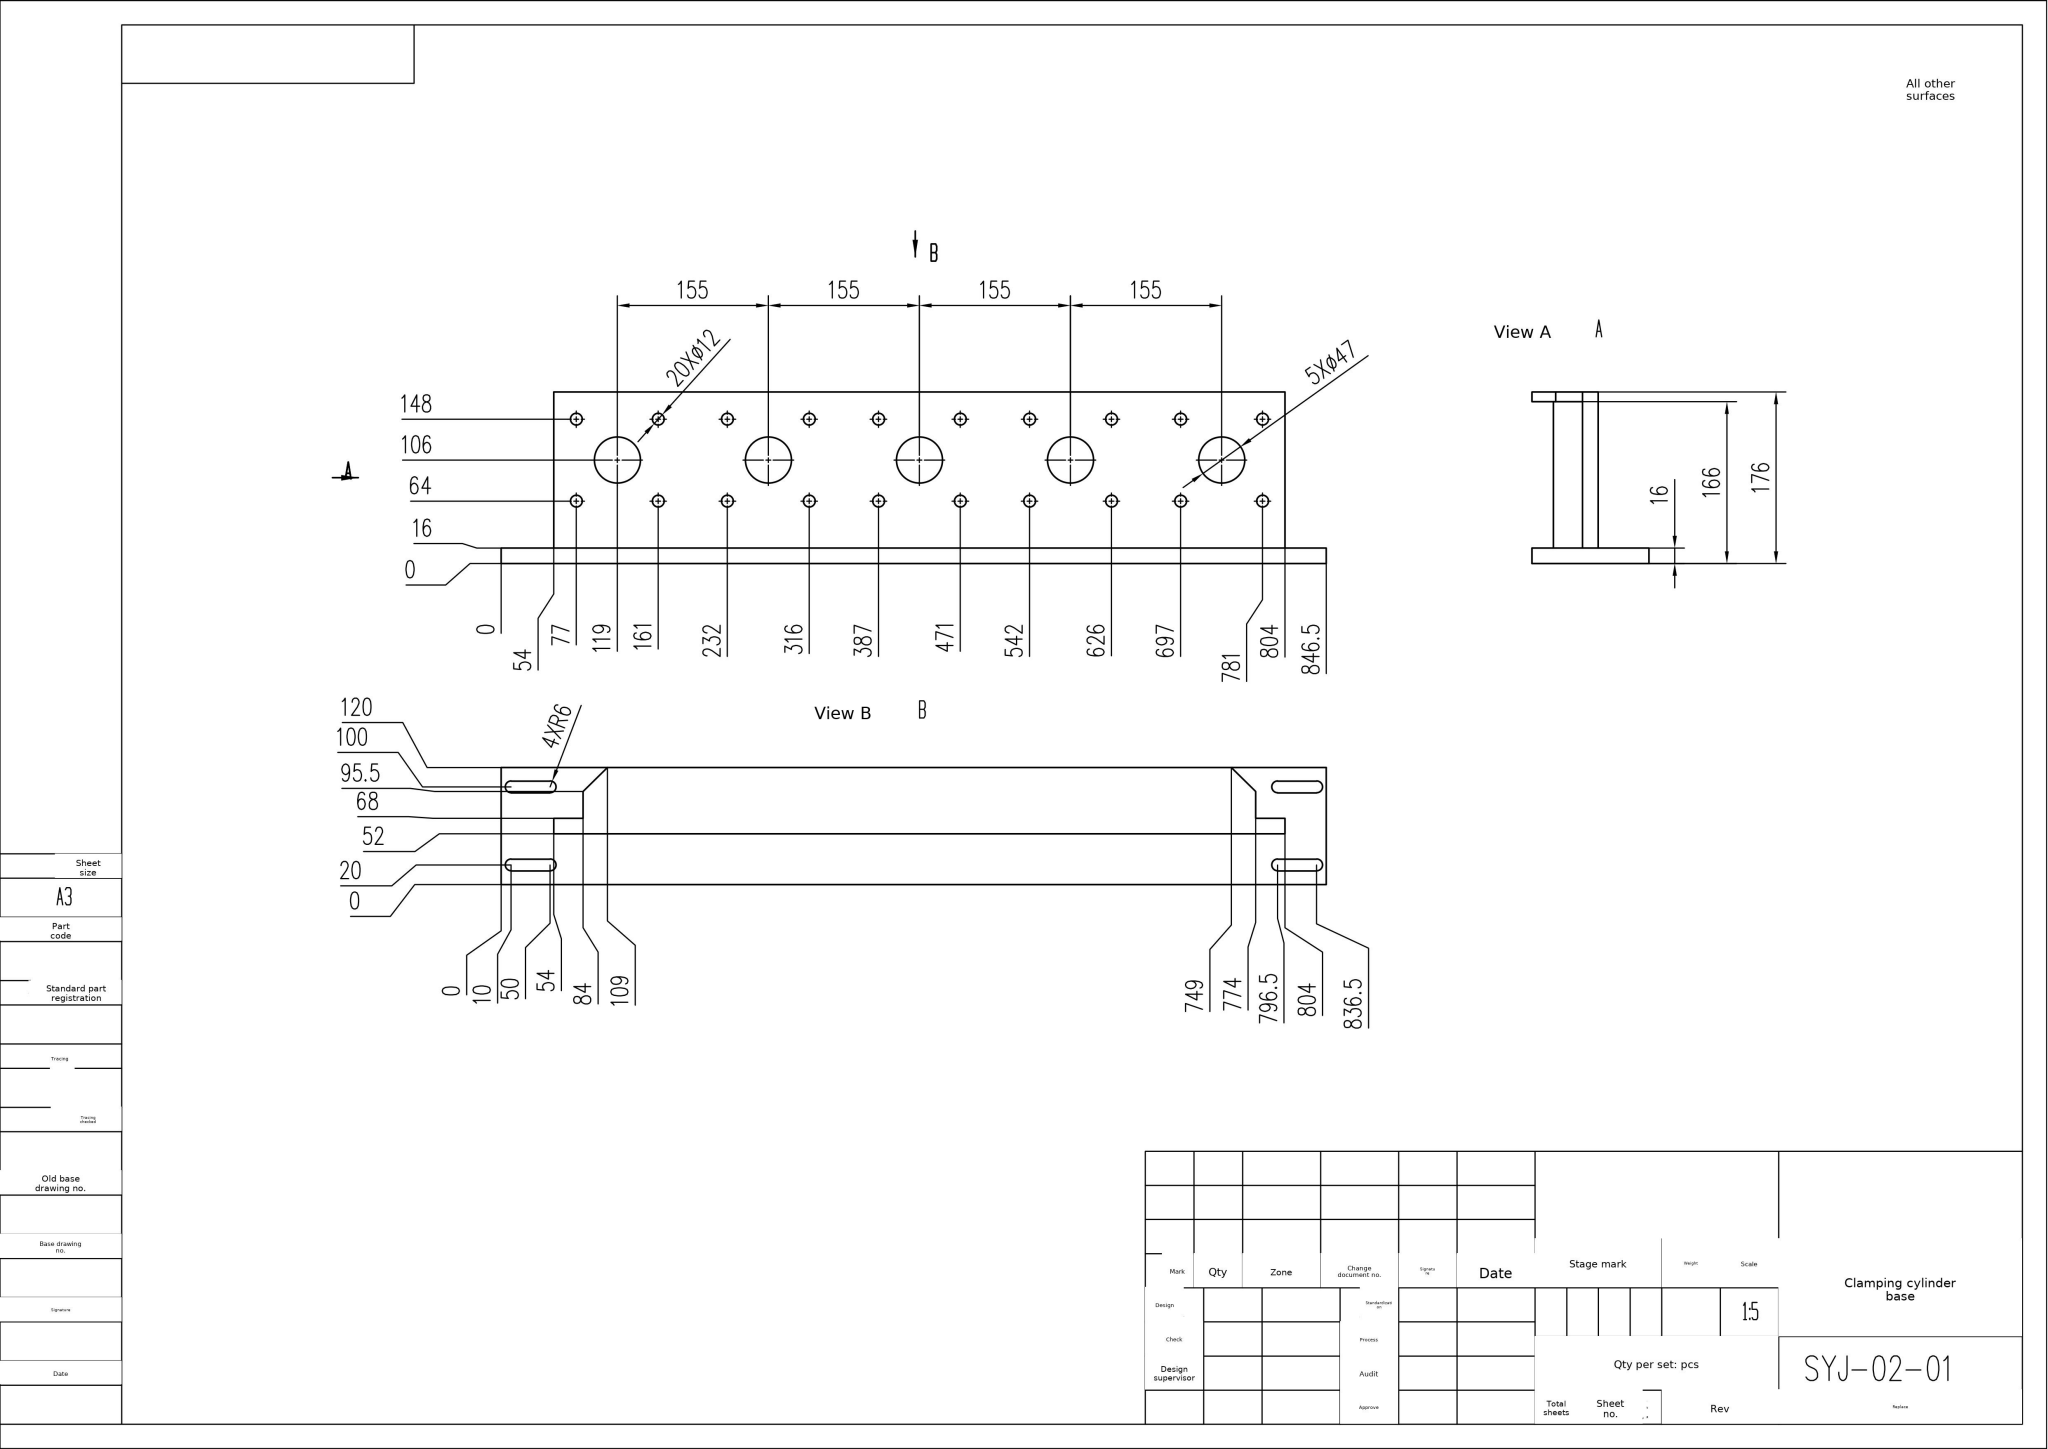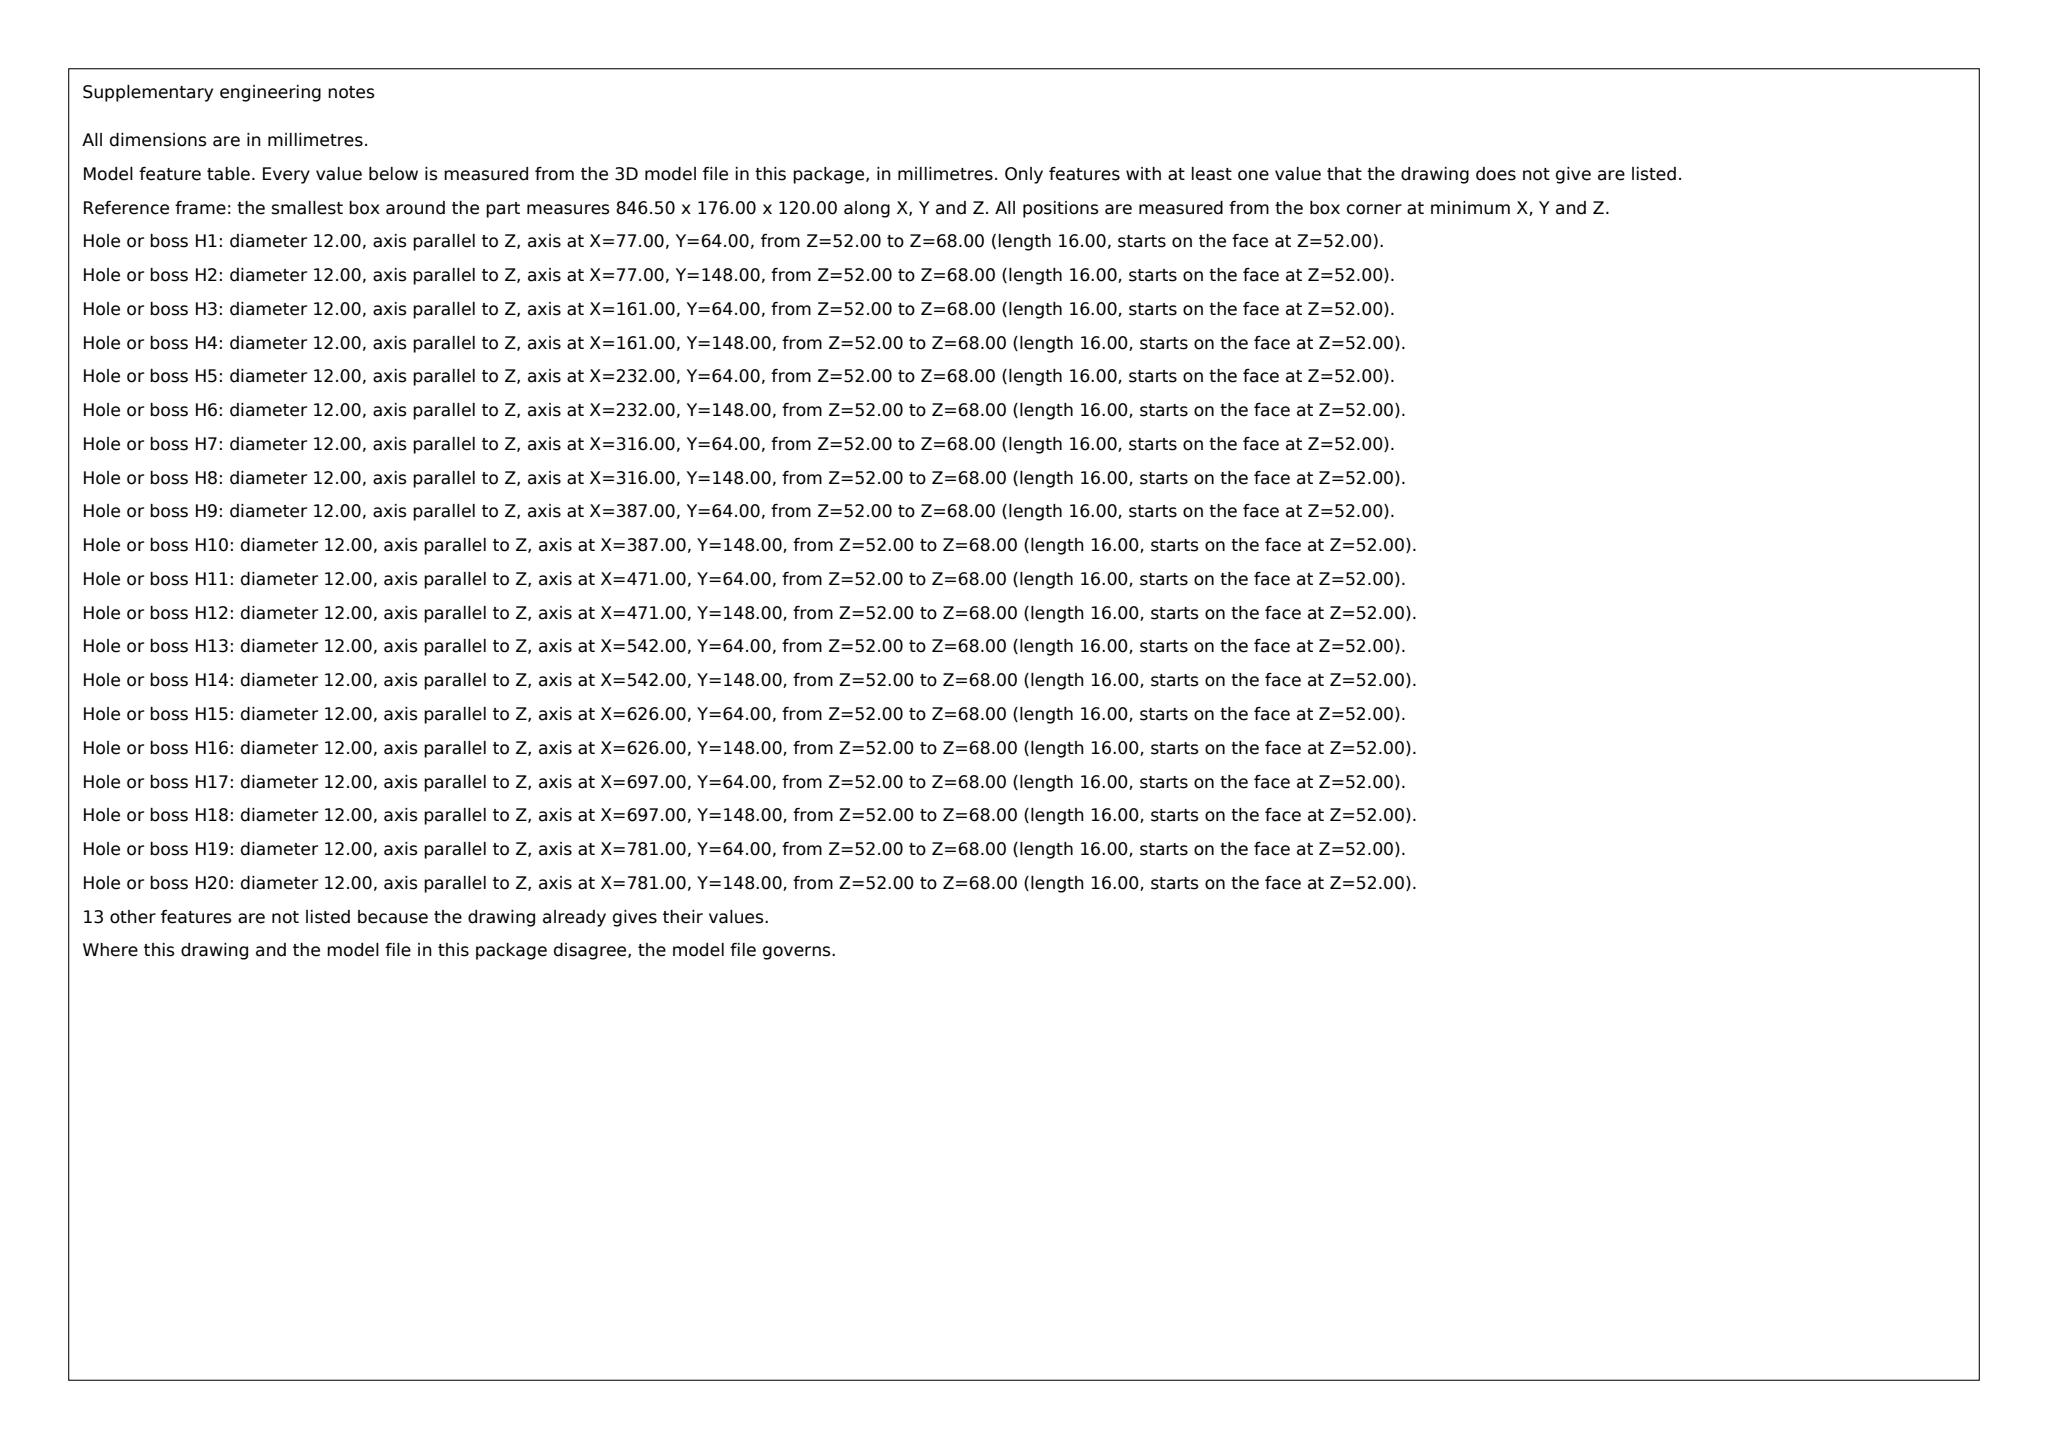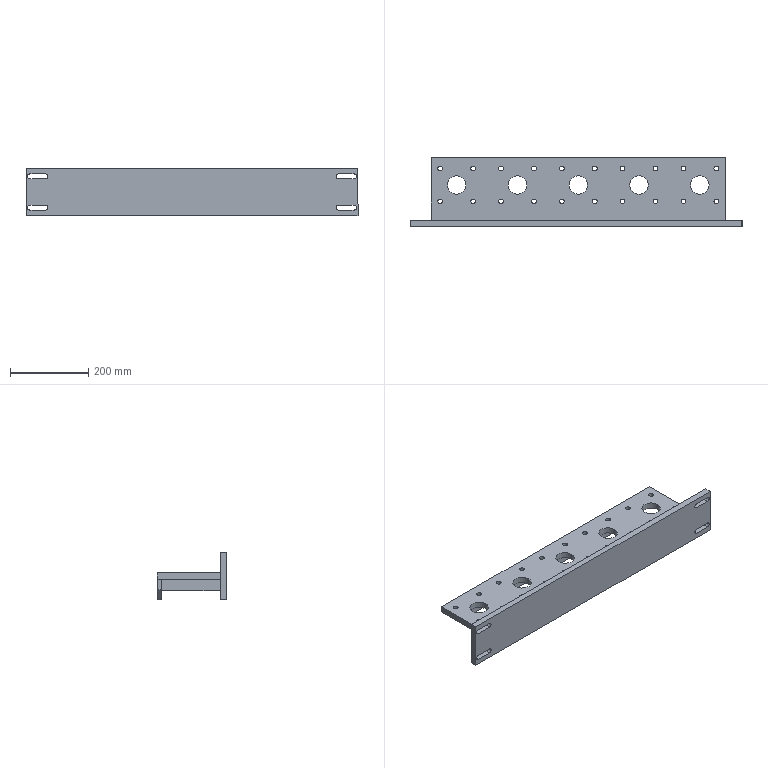Part | SolidWorks | mm | 1 solid | 91 faces | box 846.5 x 176 x 120 mm | volume 3739017 mm3 | cylinder 58 | plane 33 | commonest cylinder face diameters 12 x48 47 x10
build123d program:
from build123d import *

# Parameters (mm, degrees)
SKETCH1_W           = 810
SKETCH1_H           = 120
BOSS_EXTRUDE1_DEPTH = 16
SKETCH2_W           = 750
SKETCH2_H           = 16
BOSS_EXTRUDE2_DEPTH = 160
SKETCH5_W           = 750
SKETCH5_H           = 52
BOSS_EXTRUDE4_DEPTH = 10
CUT_EXTRUDE1_REACH  = 448.794
SKETCH6_R           = 23.5
CUT_EXTRUDE2_REACH  = 448.794
SKETCH7_R           = 6
CHAMFER1_SIZE       = 25
SKETCH9_W           = 120
SKETCH9_H           = 16
BOSS_EXTRUDE6_DEPTH = 12.5
SKETCH10_W          = 120
SKETCH10_H          = 16
BOSS_EXTRUDE7_DEPTH = 24
CUT_EXTRUDE3_DEPTH  = 16
CUT_EXTRUDE4_DEPTH  = 10
SKETCH15_W          = 6
SKETCH15_H          = 150
BOSS_EXTRUDE8_DEPTH = 30


with BuildPart() as part:
    # Sketch1 → Boss-Extrude1 (new body)
    with BuildSketch(Plane(origin=(0, 0, 0), x_dir=(1, 0, 0), z_dir=(0, 1, 0))):
        Rectangle(SKETCH1_W, SKETCH1_H)
    extrude(amount=BOSS_EXTRUDE1_DEPTH)

    # Sketch2 → Boss-Extrude2 (add)
    with BuildSketch(Plane(origin=(0, 16, 0), x_dir=(1, 0, 0), z_dir=(0, 1, 0))):
        Rectangle(SKETCH2_W, SKETCH2_H)
    extrude(amount=BOSS_EXTRUDE2_DEPTH)

    # Sketch5 → Boss-Extrude4 (add)
    with BuildSketch(Plane(origin=(0, 176, 0), x_dir=(1, 0, 0), z_dir=(0, 1, 0))):
        with Locations((0, 34)):
            Rectangle(SKETCH5_W, SKETCH5_H)
    extrude(amount=-BOSS_EXTRUDE4_DEPTH)

    # Sketch6 → Cut-Extrude1 (cut, up to next)
    with BuildSketch(Plane(origin=(0, 0, -8), x_dir=(-1, 0, 0), z_dir=(0, 0, -1)), mode=Mode.PRIVATE) as cut_extrude1_sk1:
        with Locations((0, 106)):
            Circle(SKETCH6_R)
    cut_extrude1_tool1 = extrude(cut_extrude1_sk1.sketch, amount=-CUT_EXTRUDE1_REACH, mode=Mode.PRIVATE) & part.part
    # Sketch6 → Cut-Extrude1 (cut, up to next)
    with BuildSketch(Plane(origin=(0, 0, -8), x_dir=(-1, 0, 0), z_dir=(0, 0, -1)), mode=Mode.PRIVATE) as cut_extrude1_sk2:
        with Locations((-155, 106)):
            Circle(SKETCH6_R)
    cut_extrude1_tool2 = extrude(cut_extrude1_sk2.sketch, amount=-CUT_EXTRUDE1_REACH, mode=Mode.PRIVATE) & part.part
    # Sketch6 → Cut-Extrude1 (cut, up to next)
    with BuildSketch(Plane(origin=(0, 0, -8), x_dir=(-1, 0, 0), z_dir=(0, 0, -1)), mode=Mode.PRIVATE) as cut_extrude1_sk3:
        with Locations((-310, 106)):
            Circle(SKETCH6_R)
    cut_extrude1_tool3 = extrude(cut_extrude1_sk3.sketch, amount=-CUT_EXTRUDE1_REACH, mode=Mode.PRIVATE) & part.part
    # Sketch6 → Cut-Extrude1 (cut, up to next)
    with BuildSketch(Plane(origin=(0, 0, -8), x_dir=(-1, 0, 0), z_dir=(0, 0, -1)), mode=Mode.PRIVATE) as cut_extrude1_sk4:
        with Locations((310, 106)):
            Circle(SKETCH6_R)
    cut_extrude1_tool4 = extrude(cut_extrude1_sk4.sketch, amount=-CUT_EXTRUDE1_REACH, mode=Mode.PRIVATE) & part.part
    # Sketch6 → Cut-Extrude1 (cut, up to next)
    with BuildSketch(Plane(origin=(0, 0, -8), x_dir=(-1, 0, 0), z_dir=(0, 0, -1)), mode=Mode.PRIVATE) as cut_extrude1_sk5:
        with Locations((155, 106)):
            Circle(SKETCH6_R)
    cut_extrude1_tool5 = extrude(cut_extrude1_sk5.sketch, amount=-CUT_EXTRUDE1_REACH, mode=Mode.PRIVATE) & part.part
    add(cut_extrude1_tool1.solids().sort_by_distance((0, 106, -8))[0], mode=Mode.SUBTRACT)
    add(cut_extrude1_tool2.solids().sort_by_distance((155, 106, -8))[0], mode=Mode.SUBTRACT)
    add(cut_extrude1_tool3.solids().sort_by_distance((310, 106, -8))[0], mode=Mode.SUBTRACT)
    add(cut_extrude1_tool4.solids().sort_by_distance((-310, 106, -8))[0], mode=Mode.SUBTRACT)
    add(cut_extrude1_tool5.solids().sort_by_distance((-155, 106, -8))[0], mode=Mode.SUBTRACT)

    # Sketch7 → Cut-Extrude2 (cut, up to next)
    with BuildSketch(Plane(origin=(0, 0, -8), x_dir=(-1, 0, 0), z_dir=(0, 0, -1)), mode=Mode.PRIVATE) as cut_extrude2_sk1:
        with Locations((-352, 148)):
            Circle(SKETCH7_R)
    cut_extrude2_tool1 = extrude(cut_extrude2_sk1.sketch, amount=-CUT_EXTRUDE2_REACH, mode=Mode.PRIVATE) & part.part
    # Sketch7 → Cut-Extrude2 (cut, up to next)
    with BuildSketch(Plane(origin=(0, 0, -8), x_dir=(-1, 0, 0), z_dir=(0, 0, -1)), mode=Mode.PRIVATE) as cut_extrude2_sk2:
        with Locations((-268, 148)):
            Circle(SKETCH7_R)
    cut_extrude2_tool2 = extrude(cut_extrude2_sk2.sketch, amount=-CUT_EXTRUDE2_REACH, mode=Mode.PRIVATE) & part.part
    # Sketch7 → Cut-Extrude2 (cut, up to next)
    with BuildSketch(Plane(origin=(0, 0, -8), x_dir=(-1, 0, 0), z_dir=(0, 0, -1)), mode=Mode.PRIVATE) as cut_extrude2_sk3:
        with Locations((-352, 64)):
            Circle(SKETCH7_R)
    cut_extrude2_tool3 = extrude(cut_extrude2_sk3.sketch, amount=-CUT_EXTRUDE2_REACH, mode=Mode.PRIVATE) & part.part
    # Sketch7 → Cut-Extrude2 (cut, up to next)
    with BuildSketch(Plane(origin=(0, 0, -8), x_dir=(-1, 0, 0), z_dir=(0, 0, -1)), mode=Mode.PRIVATE) as cut_extrude2_sk4:
        with Locations((-268, 64)):
            Circle(SKETCH7_R)
    cut_extrude2_tool4 = extrude(cut_extrude2_sk4.sketch, amount=-CUT_EXTRUDE2_REACH, mode=Mode.PRIVATE) & part.part
    # Sketch7 → Cut-Extrude2 (cut, up to next)
    with BuildSketch(Plane(origin=(0, 0, -8), x_dir=(-1, 0, 0), z_dir=(0, 0, -1)), mode=Mode.PRIVATE) as cut_extrude2_sk5:
        with Locations((-197, 148)):
            Circle(SKETCH7_R)
    cut_extrude2_tool5 = extrude(cut_extrude2_sk5.sketch, amount=-CUT_EXTRUDE2_REACH, mode=Mode.PRIVATE) & part.part
    # Sketch7 → Cut-Extrude2 (cut, up to next)
    with BuildSketch(Plane(origin=(0, 0, -8), x_dir=(-1, 0, 0), z_dir=(0, 0, -1)), mode=Mode.PRIVATE) as cut_extrude2_sk6:
        with Locations((-113, 148)):
            Circle(SKETCH7_R)
    cut_extrude2_tool6 = extrude(cut_extrude2_sk6.sketch, amount=-CUT_EXTRUDE2_REACH, mode=Mode.PRIVATE) & part.part
    # Sketch7 → Cut-Extrude2 (cut, up to next)
    with BuildSketch(Plane(origin=(0, 0, -8), x_dir=(-1, 0, 0), z_dir=(0, 0, -1)), mode=Mode.PRIVATE) as cut_extrude2_sk7:
        with Locations((-113, 64)):
            Circle(SKETCH7_R)
    cut_extrude2_tool7 = extrude(cut_extrude2_sk7.sketch, amount=-CUT_EXTRUDE2_REACH, mode=Mode.PRIVATE) & part.part
    # Sketch7 → Cut-Extrude2 (cut, up to next)
    with BuildSketch(Plane(origin=(0, 0, -8), x_dir=(-1, 0, 0), z_dir=(0, 0, -1)), mode=Mode.PRIVATE) as cut_extrude2_sk8:
        with Locations((-197, 64)):
            Circle(SKETCH7_R)
    cut_extrude2_tool8 = extrude(cut_extrude2_sk8.sketch, amount=-CUT_EXTRUDE2_REACH, mode=Mode.PRIVATE) & part.part
    # Sketch7 → Cut-Extrude2 (cut, up to next)
    with BuildSketch(Plane(origin=(0, 0, -8), x_dir=(-1, 0, 0), z_dir=(0, 0, -1)), mode=Mode.PRIVATE) as cut_extrude2_sk9:
        with Locations((-42, 148)):
            Circle(SKETCH7_R)
    cut_extrude2_tool9 = extrude(cut_extrude2_sk9.sketch, amount=-CUT_EXTRUDE2_REACH, mode=Mode.PRIVATE) & part.part
    # Sketch7 → Cut-Extrude2 (cut, up to next)
    with BuildSketch(Plane(origin=(0, 0, -8), x_dir=(-1, 0, 0), z_dir=(0, 0, -1)), mode=Mode.PRIVATE) as cut_extrude2_sk10:
        with Locations((42, 148)):
            Circle(SKETCH7_R)
    cut_extrude2_tool10 = extrude(cut_extrude2_sk10.sketch, amount=-CUT_EXTRUDE2_REACH, mode=Mode.PRIVATE) & part.part
    # Sketch7 → Cut-Extrude2 (cut, up to next)
    with BuildSketch(Plane(origin=(0, 0, -8), x_dir=(-1, 0, 0), z_dir=(0, 0, -1)), mode=Mode.PRIVATE) as cut_extrude2_sk11:
        with Locations((42, 64)):
            Circle(SKETCH7_R)
    cut_extrude2_tool11 = extrude(cut_extrude2_sk11.sketch, amount=-CUT_EXTRUDE2_REACH, mode=Mode.PRIVATE) & part.part
    # Sketch7 → Cut-Extrude2 (cut, up to next)
    with BuildSketch(Plane(origin=(0, 0, -8), x_dir=(-1, 0, 0), z_dir=(0, 0, -1)), mode=Mode.PRIVATE) as cut_extrude2_sk12:
        with Locations((-42, 64)):
            Circle(SKETCH7_R)
    cut_extrude2_tool12 = extrude(cut_extrude2_sk12.sketch, amount=-CUT_EXTRUDE2_REACH, mode=Mode.PRIVATE) & part.part
    # Sketch7 → Cut-Extrude2 (cut, up to next)
    with BuildSketch(Plane(origin=(0, 0, -8), x_dir=(-1, 0, 0), z_dir=(0, 0, -1)), mode=Mode.PRIVATE) as cut_extrude2_sk13:
        with Locations((113, 148)):
            Circle(SKETCH7_R)
    cut_extrude2_tool13 = extrude(cut_extrude2_sk13.sketch, amount=-CUT_EXTRUDE2_REACH, mode=Mode.PRIVATE) & part.part
    # Sketch7 → Cut-Extrude2 (cut, up to next)
    with BuildSketch(Plane(origin=(0, 0, -8), x_dir=(-1, 0, 0), z_dir=(0, 0, -1)), mode=Mode.PRIVATE) as cut_extrude2_sk14:
        with Locations((197, 148)):
            Circle(SKETCH7_R)
    cut_extrude2_tool14 = extrude(cut_extrude2_sk14.sketch, amount=-CUT_EXTRUDE2_REACH, mode=Mode.PRIVATE) & part.part
    # Sketch7 → Cut-Extrude2 (cut, up to next)
    with BuildSketch(Plane(origin=(0, 0, -8), x_dir=(-1, 0, 0), z_dir=(0, 0, -1)), mode=Mode.PRIVATE) as cut_extrude2_sk15:
        with Locations((197, 64)):
            Circle(SKETCH7_R)
    cut_extrude2_tool15 = extrude(cut_extrude2_sk15.sketch, amount=-CUT_EXTRUDE2_REACH, mode=Mode.PRIVATE) & part.part
    # Sketch7 → Cut-Extrude2 (cut, up to next)
    with BuildSketch(Plane(origin=(0, 0, -8), x_dir=(-1, 0, 0), z_dir=(0, 0, -1)), mode=Mode.PRIVATE) as cut_extrude2_sk16:
        with Locations((113, 64)):
            Circle(SKETCH7_R)
    cut_extrude2_tool16 = extrude(cut_extrude2_sk16.sketch, amount=-CUT_EXTRUDE2_REACH, mode=Mode.PRIVATE) & part.part
    # Sketch7 → Cut-Extrude2 (cut, up to next)
    with BuildSketch(Plane(origin=(0, 0, -8), x_dir=(-1, 0, 0), z_dir=(0, 0, -1)), mode=Mode.PRIVATE) as cut_extrude2_sk17:
        with Locations((268, 148)):
            Circle(SKETCH7_R)
    cut_extrude2_tool17 = extrude(cut_extrude2_sk17.sketch, amount=-CUT_EXTRUDE2_REACH, mode=Mode.PRIVATE) & part.part
    # Sketch7 → Cut-Extrude2 (cut, up to next)
    with BuildSketch(Plane(origin=(0, 0, -8), x_dir=(-1, 0, 0), z_dir=(0, 0, -1)), mode=Mode.PRIVATE) as cut_extrude2_sk18:
        with Locations((352, 148)):
            Circle(SKETCH7_R)
    cut_extrude2_tool18 = extrude(cut_extrude2_sk18.sketch, amount=-CUT_EXTRUDE2_REACH, mode=Mode.PRIVATE) & part.part
    # Sketch7 → Cut-Extrude2 (cut, up to next)
    with BuildSketch(Plane(origin=(0, 0, -8), x_dir=(-1, 0, 0), z_dir=(0, 0, -1)), mode=Mode.PRIVATE) as cut_extrude2_sk19:
        with Locations((352, 64)):
            Circle(SKETCH7_R)
    cut_extrude2_tool19 = extrude(cut_extrude2_sk19.sketch, amount=-CUT_EXTRUDE2_REACH, mode=Mode.PRIVATE) & part.part
    # Sketch7 → Cut-Extrude2 (cut, up to next)
    with BuildSketch(Plane(origin=(0, 0, -8), x_dir=(-1, 0, 0), z_dir=(0, 0, -1)), mode=Mode.PRIVATE) as cut_extrude2_sk20:
        with Locations((268, 64)):
            Circle(SKETCH7_R)
    cut_extrude2_tool20 = extrude(cut_extrude2_sk20.sketch, amount=-CUT_EXTRUDE2_REACH, mode=Mode.PRIVATE) & part.part
    add(cut_extrude2_tool1.solids().sort_by_distance((352, 148, -8))[0], mode=Mode.SUBTRACT)
    add(cut_extrude2_tool2.solids().sort_by_distance((268, 148, -8))[0], mode=Mode.SUBTRACT)
    add(cut_extrude2_tool3.solids().sort_by_distance((352, 64, -8))[0], mode=Mode.SUBTRACT)
    add(cut_extrude2_tool4.solids().sort_by_distance((268, 64, -8))[0], mode=Mode.SUBTRACT)
    add(cut_extrude2_tool5.solids().sort_by_distance((197, 148, -8))[0], mode=Mode.SUBTRACT)
    add(cut_extrude2_tool6.solids().sort_by_distance((113, 148, -8))[0], mode=Mode.SUBTRACT)
    add(cut_extrude2_tool7.solids().sort_by_distance((113, 64, -8))[0], mode=Mode.SUBTRACT)
    add(cut_extrude2_tool8.solids().sort_by_distance((197, 64, -8))[0], mode=Mode.SUBTRACT)
    add(cut_extrude2_tool9.solids().sort_by_distance((42, 148, -8))[0], mode=Mode.SUBTRACT)
    add(cut_extrude2_tool10.solids().sort_by_distance((-42, 148, -8))[0], mode=Mode.SUBTRACT)
    add(cut_extrude2_tool11.solids().sort_by_distance((-42, 64, -8))[0], mode=Mode.SUBTRACT)
    add(cut_extrude2_tool12.solids().sort_by_distance((42, 64, -8))[0], mode=Mode.SUBTRACT)
    add(cut_extrude2_tool13.solids().sort_by_distance((-113, 148, -8))[0], mode=Mode.SUBTRACT)
    add(cut_extrude2_tool14.solids().sort_by_distance((-197, 148, -8))[0], mode=Mode.SUBTRACT)
    add(cut_extrude2_tool15.solids().sort_by_distance((-197, 64, -8))[0], mode=Mode.SUBTRACT)
    add(cut_extrude2_tool16.solids().sort_by_distance((-113, 64, -8))[0], mode=Mode.SUBTRACT)
    add(cut_extrude2_tool17.solids().sort_by_distance((-268, 148, -8))[0], mode=Mode.SUBTRACT)
    add(cut_extrude2_tool18.solids().sort_by_distance((-352, 148, -8))[0], mode=Mode.SUBTRACT)
    add(cut_extrude2_tool19.solids().sort_by_distance((-352, 64, -8))[0], mode=Mode.SUBTRACT)
    add(cut_extrude2_tool20.solids().sort_by_distance((-268, 64, -8))[0], mode=Mode.SUBTRACT)

    # Chamfer1
    chamfer1_edges = [part.edges().sort_by_distance(p)[0] for p in [
        (-375, 171, -60),
        (375, 171, -60),
    ]]
    chamfer(chamfer1_edges, length=CHAMFER1_SIZE)

    # Sketch9 → Boss-Extrude6 (add)
    with BuildSketch(Plane(origin=(405, 0, 0), x_dir=(0, 0, -1), z_dir=(1, 0, 0))):
        with Locations((0, 8)):
            Rectangle(SKETCH9_W, SKETCH9_H)
    extrude(amount=BOSS_EXTRUDE6_DEPTH)

    # Sketch10 → Boss-Extrude7 (add)
    with BuildSketch(Plane.ZY.offset(405)):
        with Locations((0, 8)):
            Rectangle(SKETCH10_W, SKETCH10_H)
    extrude(amount=BOSS_EXTRUDE7_DEPTH)

    # Sketch11 → Cut-Extrude3 (cut)
    with BuildSketch(Plane(origin=(0, 16, 0), x_dir=(1, 0, 0), z_dir=(0, 1, 0))):
        with BuildLine():
            Line((-419, 46), (-379, 46))
            ThreePointArc((-379, 46), (-373, 40), (-379, 34))
            Line((-379, 34), (-419, 34))
            ThreePointArc((-419, 34), (-425, 40), (-419, 46))
        make_face()
        with BuildLine():
            Line((-419, -46), (-379, -46))
            ThreePointArc((-379, -46), (-373, -40), (-379, -34))
            Line((-379, -34), (-419, -34))
            ThreePointArc((-419, -34), (-425, -40), (-419, -46))
        make_face()
        with BuildLine():
            Line((407.5, -46), (367.5, -46))
            ThreePointArc((367.5, -46), (361.5, -40), (367.5, -34))
            Line((367.5, -34), (407.5, -34))
            ThreePointArc((407.5, -34), (413.5, -40), (407.5, -46))
        make_face()
        with BuildLine():
            Line((407.5, 46), (367.5, 46))
            ThreePointArc((367.5, 46), (361.5, 40), (367.5, 34))
            Line((367.5, 34), (407.5, 34))
            ThreePointArc((407.5, 34), (413.5, 40), (407.5, 46))
        make_face()
    extrude(amount=-CUT_EXTRUDE3_DEPTH, mode=Mode.SUBTRACT)

    # Sketch14 → Cut-Extrude4 (cut)
    with BuildSketch(Plane(origin=(0, 176, 0), x_dir=(1, 0, 0), z_dir=(0, 1, 0))):
        Polygon((-320, 60), (-345, 35.528), (-345, 8), (-375, 8), (-375, 35.528), (-350, 60), align=None)
        Polygon((350, 60), (320, 60), (345, 35.528), (345, 8), (375, 8), (375, 35.528), align=None)
    extrude(amount=-CUT_EXTRUDE4_DEPTH, mode=Mode.SUBTRACT)

    # Sketch15 → Boss-Extrude8 (add)
    with BuildSketch(Plane(origin=(0, 0, -8), x_dir=(-1, 0, 0), z_dir=(0, 0, -1))):
        with Locations((-232.5, 91)):
            Rectangle(SKETCH15_W, SKETCH15_H)
        with Locations((232.5, 91)):
            Rectangle(SKETCH15_W, SKETCH15_H)
    extrude(amount=BOSS_EXTRUDE8_DEPTH)


solid = part.part